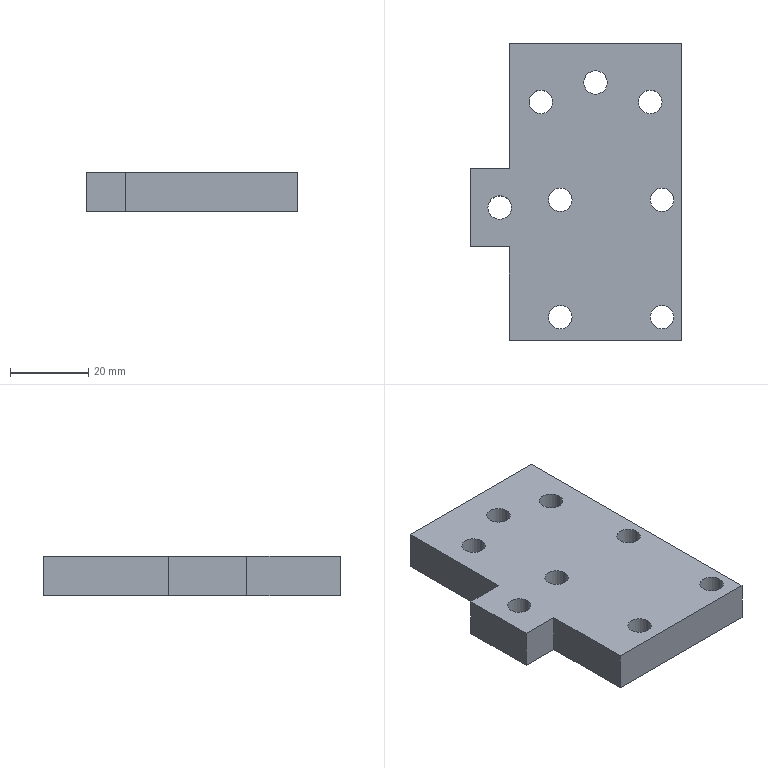Component | SolidWorks | SupportPlate-1 | 1 solid | 26 faces | box 54 x 76 x 10 mm | volume 33178 mm3 | cylinder 16 | plane 10 | commonest cylinder face diameters 6 x16
build123d program:
from build123d import *

# Parameters (mm, degrees)
SKETCH1_R           = 3
BOSS_EXTRUDE1_DEPTH = 10


with BuildPart() as part:
    # Sketch1 → Boss-Extrude1 (new body)
    with BuildSketch(Plane(origin=(0, 0, -5), x_dir=(-1, 0, 0), z_dir=(0, 0, -1))):
        Polygon((22, -9), (32, -9), (32, 11), (22, 11), (22, 43), (-22, 43), (-22, -33), (22, -33), align=None)
        with Locations(Location((0, 33, 0), (0, 0, 180))):
            Circle(SKETCH1_R, mode=Mode.SUBTRACT)
        with Locations(Location((14, 28, 0), (0, 0, 180))):
            Circle(SKETCH1_R, mode=Mode.SUBTRACT)
        with Locations(Location((9, -27, 0), (0, 0, 180))):
            Circle(SKETCH1_R, mode=Mode.SUBTRACT)
        with Locations(Location((9, 3, 0), (0, 0, 180))):
            Circle(SKETCH1_R, mode=Mode.SUBTRACT)
        with Locations(Location((-17, 3, 0), (0, 0, 180))):
            Circle(SKETCH1_R, mode=Mode.SUBTRACT)
        with Locations(Location((-17, -27, 0), (0, 0, 180))):
            Circle(SKETCH1_R, mode=Mode.SUBTRACT)
        with Locations(Location((-14, 28, 0), (0, 0, 180))):
            Circle(SKETCH1_R, mode=Mode.SUBTRACT)
        with Locations(Location((24.5, 1, 0), (0, 0, 180))):
            Circle(SKETCH1_R, mode=Mode.SUBTRACT)
    extrude(amount=-BOSS_EXTRUDE1_DEPTH)


solid = part.part

# Placed as in the assembly
solid = solid.moved(Location((196.793, 568, -207.5), (0, 0, 0)))
STEP:
#1=COLOUR_RGB('',0.7922,0.8196,0.9333);
#2=FILL_AREA_STYLE_COLOUR('',#1);
#3=FILL_AREA_STYLE('',(#2));
#4=SURFACE_STYLE_FILL_AREA(#3);
#5=SURFACE_SIDE_STYLE('',(#4));
#6=SURFACE_STYLE_USAGE(.BOTH.,#5);
#7=PRESENTATION_STYLE_ASSIGNMENT((#6));
#8=CARTESIAN_POINT('',(6.901,22.402,-7.972));
#9=VERTEX_POINT('',#8);
#10=CARTESIAN_POINT('',(6.665,22.402,-7.972));
#11=VERTEX_POINT('',#10);
#12=CARTESIAN_POINT('',(6.783,22.402,-7.972));
#13=DIRECTION('',(0.,0.,-1.));
#14=DIRECTION('',(1.,0.,0.));
#15=AXIS2_PLACEMENT_3D('',#12,#13,#14);
#16=CIRCLE('',#15,0.1181);
#17=EDGE_CURVE('',#9,#11,#16,.T.);
#18=ORIENTED_EDGE('',*,*,#17,.F.);
#19=CARTESIAN_POINT('',(6.901,22.402,-8.366));
#20=VERTEX_POINT('',#19);
#21=CARTESIAN_POINT('',(6.901,22.402,-7.972));
#22=DIRECTION('',(0.,0.,-1.));
#23=VECTOR('',#22,39.37);
#24=LINE('',#21,#23);
#25=EDGE_CURVE('',#9,#20,#24,.T.);
#26=ORIENTED_EDGE('',*,*,#25,.T.);
#27=CARTESIAN_POINT('',(6.665,22.402,-8.366));
#28=VERTEX_POINT('',#27);
#29=CARTESIAN_POINT('',(6.783,22.402,-8.366));
#30=DIRECTION('',(0.,0.,-1.));
#31=DIRECTION('',(1.,0.,0.));
#32=AXIS2_PLACEMENT_3D('',#29,#30,#31);
#33=CIRCLE('',#32,0.1181);
#34=EDGE_CURVE('',#20,#28,#33,.T.);
#35=ORIENTED_EDGE('',*,*,#34,.T.);
#36=CARTESIAN_POINT('',(6.665,22.402,-7.972));
#37=DIRECTION('',(0.,0.,-1.));
#38=VECTOR('',#37,39.37);
#39=LINE('',#36,#38);
#40=EDGE_CURVE('',#11,#28,#39,.T.);
#41=ORIENTED_EDGE('',*,*,#40,.F.);
#42=EDGE_LOOP('',(#18,#26,#35,#41));
#43=FACE_OUTER_BOUND('',#42,.T.);
#44=CARTESIAN_POINT('',(6.783,22.402,-7.972));
#45=DIRECTION('',(0.,0.,-1.));
#46=DIRECTION('',(-1.,0.,0.));
#47=AXIS2_PLACEMENT_3D('',#44,#45,#46);
#48=CYLINDRICAL_SURFACE('',#47,0.1181);
#49=ADVANCED_FACE('',(#43),#48,.F.);
#50=CARTESIAN_POINT('',(8.417,23.465,-7.972));
#51=VERTEX_POINT('',#50);
#52=CARTESIAN_POINT('',(8.181,23.465,-7.972));
#53=VERTEX_POINT('',#52);
#54=CARTESIAN_POINT('',(8.299,23.465,-7.972));
#55=DIRECTION('',(0.,0.,-1.));
#56=DIRECTION('',(1.,0.,0.));
#57=AXIS2_PLACEMENT_3D('',#54,#55,#56);
#58=CIRCLE('',#57,0.1181);
#59=EDGE_CURVE('',#51,#53,#58,.T.);
#60=ORIENTED_EDGE('',*,*,#59,.F.);
#61=CARTESIAN_POINT('',(8.417,23.465,-8.366));
#62=VERTEX_POINT('',#61);
#63=CARTESIAN_POINT('',(8.417,23.465,-7.972));
#64=DIRECTION('',(0.,0.,-1.));
#65=VECTOR('',#64,39.37);
#66=LINE('',#63,#65);
#67=EDGE_CURVE('',#51,#62,#66,.T.);
#68=ORIENTED_EDGE('',*,*,#67,.T.);
#69=CARTESIAN_POINT('',(8.181,23.465,-8.366));
#70=VERTEX_POINT('',#69);
#71=CARTESIAN_POINT('',(8.299,23.465,-8.366));
#72=DIRECTION('',(0.,0.,-1.));
#73=DIRECTION('',(1.,0.,0.));
#74=AXIS2_PLACEMENT_3D('',#71,#72,#73);
#75=CIRCLE('',#74,0.1181);
#76=EDGE_CURVE('',#62,#70,#75,.T.);
#77=ORIENTED_EDGE('',*,*,#76,.T.);
#78=CARTESIAN_POINT('',(8.181,23.465,-7.972));
#79=DIRECTION('',(0.,0.,-1.));
#80=VECTOR('',#79,39.37);
#81=LINE('',#78,#80);
#82=EDGE_CURVE('',#53,#70,#81,.T.);
#83=ORIENTED_EDGE('',*,*,#82,.F.);
#84=EDGE_LOOP('',(#60,#68,#77,#83));
#85=FACE_OUTER_BOUND('',#84,.T.);
#86=CARTESIAN_POINT('',(8.299,23.465,-7.972));
#87=DIRECTION('',(0.,0.,-1.));
#88=DIRECTION('',(-1.,0.,0.));
#89=AXIS2_PLACEMENT_3D('',#86,#87,#88);
#90=CYLINDRICAL_SURFACE('',#89,0.1181);
#91=ADVANCED_FACE('',(#85),#90,.F.);
#92=CARTESIAN_POINT('',(8.535,21.299,-7.972));
#93=VERTEX_POINT('',#92);
#94=CARTESIAN_POINT('',(8.299,21.299,-7.972));
#95=VERTEX_POINT('',#94);
#96=CARTESIAN_POINT('',(8.417,21.299,-7.972));
#97=DIRECTION('',(0.,0.,-1.));
#98=DIRECTION('',(1.,0.,0.));
#99=AXIS2_PLACEMENT_3D('',#96,#97,#98);
#100=CIRCLE('',#99,0.1181);
#101=EDGE_CURVE('',#93,#95,#100,.T.);
#102=ORIENTED_EDGE('',*,*,#101,.F.);
#103=CARTESIAN_POINT('',(8.535,21.299,-8.366));
#104=VERTEX_POINT('',#103);
#105=CARTESIAN_POINT('',(8.535,21.299,-7.972));
#106=DIRECTION('',(0.,0.,-1.));
#107=VECTOR('',#106,39.37);
#108=LINE('',#105,#107);
#109=EDGE_CURVE('',#93,#104,#108,.T.);
#110=ORIENTED_EDGE('',*,*,#109,.T.);
#111=CARTESIAN_POINT('',(8.299,21.299,-8.366));
#112=VERTEX_POINT('',#111);
#113=CARTESIAN_POINT('',(8.417,21.299,-8.366));
#114=DIRECTION('',(0.,0.,-1.));
#115=DIRECTION('',(1.,0.,0.));
#116=AXIS2_PLACEMENT_3D('',#113,#114,#115);
#117=CIRCLE('',#116,0.1181);
#118=EDGE_CURVE('',#104,#112,#117,.T.);
#119=ORIENTED_EDGE('',*,*,#118,.T.);
#120=CARTESIAN_POINT('',(8.299,21.299,-7.972));
#121=DIRECTION('',(0.,0.,-1.));
#122=VECTOR('',#121,39.37);
#123=LINE('',#120,#122);
#124=EDGE_CURVE('',#95,#112,#123,.T.);
#125=ORIENTED_EDGE('',*,*,#124,.F.);
#126=EDGE_LOOP('',(#102,#110,#119,#125));
#127=FACE_OUTER_BOUND('',#126,.T.);
#128=CARTESIAN_POINT('',(8.417,21.299,-7.972));
#129=DIRECTION('',(0.,0.,-1.));
#130=DIRECTION('',(-1.,0.,0.));
#131=AXIS2_PLACEMENT_3D('',#128,#129,#130);
#132=CYLINDRICAL_SURFACE('',#131,0.1181);
#133=ADVANCED_FACE('',(#127),#132,.F.);
#134=CARTESIAN_POINT('',(8.535,22.48,-7.972));
#135=VERTEX_POINT('',#134);
#136=CARTESIAN_POINT('',(8.299,22.48,-7.972));
#137=VERTEX_POINT('',#136);
#138=CARTESIAN_POINT('',(8.417,22.48,-7.972));
#139=DIRECTION('',(0.,0.,-1.));
#140=DIRECTION('',(1.,0.,0.));
#141=AXIS2_PLACEMENT_3D('',#138,#139,#140);
#142=CIRCLE('',#141,0.1181);
#143=EDGE_CURVE('',#135,#137,#142,.T.);
#144=ORIENTED_EDGE('',*,*,#143,.F.);
#145=CARTESIAN_POINT('',(8.535,22.48,-8.366));
#146=VERTEX_POINT('',#145);
#147=CARTESIAN_POINT('',(8.535,22.48,-7.972));
#148=DIRECTION('',(0.,0.,-1.));
#149=VECTOR('',#148,39.37);
#150=LINE('',#147,#149);
#151=EDGE_CURVE('',#135,#146,#150,.T.);
#152=ORIENTED_EDGE('',*,*,#151,.T.);
#153=CARTESIAN_POINT('',(8.299,22.48,-8.366));
#154=VERTEX_POINT('',#153);
#155=CARTESIAN_POINT('',(8.417,22.48,-8.366));
#156=DIRECTION('',(0.,0.,-1.));
#157=DIRECTION('',(1.,0.,0.));
#158=AXIS2_PLACEMENT_3D('',#155,#156,#157);
#159=CIRCLE('',#158,0.1181);
#160=EDGE_CURVE('',#146,#154,#159,.T.);
#161=ORIENTED_EDGE('',*,*,#160,.T.);
#162=CARTESIAN_POINT('',(8.299,22.48,-7.972));
#163=DIRECTION('',(0.,0.,-1.));
#164=VECTOR('',#163,39.37);
#165=LINE('',#162,#164);
#166=EDGE_CURVE('',#137,#154,#165,.T.);
#167=ORIENTED_EDGE('',*,*,#166,.F.);
#168=EDGE_LOOP('',(#144,#152,#161,#167));
#169=FACE_OUTER_BOUND('',#168,.T.);
#170=CARTESIAN_POINT('',(8.417,22.48,-7.972));
#171=DIRECTION('',(0.,0.,-1.));
#172=DIRECTION('',(-1.,0.,0.));
#173=AXIS2_PLACEMENT_3D('',#170,#171,#172);
#174=CYLINDRICAL_SURFACE('',#173,0.1181);
#175=ADVANCED_FACE('',(#169),#174,.F.);
#176=CARTESIAN_POINT('',(7.512,22.48,-7.972));
#177=VERTEX_POINT('',#176);
#178=CARTESIAN_POINT('',(7.275,22.48,-7.972));
#179=VERTEX_POINT('',#178);
#180=CARTESIAN_POINT('',(7.393,22.48,-7.972));
#181=DIRECTION('',(0.,0.,-1.));
#182=DIRECTION('',(1.,0.,0.));
#183=AXIS2_PLACEMENT_3D('',#180,#181,#182);
#184=CIRCLE('',#183,0.1181);
#185=EDGE_CURVE('',#177,#179,#184,.T.);
#186=ORIENTED_EDGE('',*,*,#185,.F.);
#187=CARTESIAN_POINT('',(7.512,22.48,-8.366));
#188=VERTEX_POINT('',#187);
#189=CARTESIAN_POINT('',(7.512,22.48,-7.972));
#190=DIRECTION('',(0.,0.,-1.));
#191=VECTOR('',#190,39.37);
#192=LINE('',#189,#191);
#193=EDGE_CURVE('',#177,#188,#192,.T.);
#194=ORIENTED_EDGE('',*,*,#193,.T.);
#195=CARTESIAN_POINT('',(7.275,22.48,-8.366));
#196=VERTEX_POINT('',#195);
#197=CARTESIAN_POINT('',(7.393,22.48,-8.366));
#198=DIRECTION('',(0.,0.,-1.));
#199=DIRECTION('',(1.,0.,0.));
#200=AXIS2_PLACEMENT_3D('',#197,#198,#199);
#201=CIRCLE('',#200,0.1181);
#202=EDGE_CURVE('',#188,#196,#201,.T.);
#203=ORIENTED_EDGE('',*,*,#202,.T.);
#204=CARTESIAN_POINT('',(7.275,22.48,-7.972));
#205=DIRECTION('',(0.,0.,-1.));
#206=VECTOR('',#205,39.37);
#207=LINE('',#204,#206);
#208=EDGE_CURVE('',#179,#196,#207,.T.);
#209=ORIENTED_EDGE('',*,*,#208,.F.);
#210=EDGE_LOOP('',(#186,#194,#203,#209));
#211=FACE_OUTER_BOUND('',#210,.T.);
#212=CARTESIAN_POINT('',(7.393,22.48,-7.972));
#213=DIRECTION('',(0.,0.,-1.));
#214=DIRECTION('',(-1.,0.,0.));
#215=AXIS2_PLACEMENT_3D('',#212,#213,#214);
#216=CYLINDRICAL_SURFACE('',#215,0.1181);
#217=ADVANCED_FACE('',(#211),#216,.F.);
#218=CARTESIAN_POINT('',(7.512,21.299,-7.972));
#219=VERTEX_POINT('',#218);
#220=CARTESIAN_POINT('',(7.275,21.299,-7.972));
#221=VERTEX_POINT('',#220);
#222=CARTESIAN_POINT('',(7.393,21.299,-7.972));
#223=DIRECTION('',(0.,0.,-1.));
#224=DIRECTION('',(1.,0.,0.));
#225=AXIS2_PLACEMENT_3D('',#222,#223,#224);
#226=CIRCLE('',#225,0.1181);
#227=EDGE_CURVE('',#219,#221,#226,.T.);
#228=ORIENTED_EDGE('',*,*,#227,.F.);
#229=CARTESIAN_POINT('',(7.512,21.299,-8.366));
#230=VERTEX_POINT('',#229);
#231=CARTESIAN_POINT('',(7.512,21.299,-7.972));
#232=DIRECTION('',(0.,0.,-1.));
#233=VECTOR('',#232,39.37);
#234=LINE('',#231,#233);
#235=EDGE_CURVE('',#219,#230,#234,.T.);
#236=ORIENTED_EDGE('',*,*,#235,.T.);
#237=CARTESIAN_POINT('',(7.275,21.299,-8.366));
#238=VERTEX_POINT('',#237);
#239=CARTESIAN_POINT('',(7.393,21.299,-8.366));
#240=DIRECTION('',(0.,0.,-1.));
#241=DIRECTION('',(1.,0.,0.));
#242=AXIS2_PLACEMENT_3D('',#239,#240,#241);
#243=CIRCLE('',#242,0.1181);
#244=EDGE_CURVE('',#230,#238,#243,.T.);
#245=ORIENTED_EDGE('',*,*,#244,.T.);
#246=CARTESIAN_POINT('',(7.275,21.299,-7.972));
#247=DIRECTION('',(0.,0.,-1.));
#248=VECTOR('',#247,39.37);
#249=LINE('',#246,#248);
#250=EDGE_CURVE('',#221,#238,#249,.T.);
#251=ORIENTED_EDGE('',*,*,#250,.F.);
#252=EDGE_LOOP('',(#228,#236,#245,#251));
#253=FACE_OUTER_BOUND('',#252,.T.);
#254=CARTESIAN_POINT('',(7.393,21.299,-7.972));
#255=DIRECTION('',(0.,0.,-1.));
#256=DIRECTION('',(-1.,0.,0.));
#257=AXIS2_PLACEMENT_3D('',#254,#255,#256);
#258=CYLINDRICAL_SURFACE('',#257,0.1181);
#259=ADVANCED_FACE('',(#253),#258,.F.);
#260=CARTESIAN_POINT('',(7.315,23.465,-7.972));
#261=VERTEX_POINT('',#260);
#262=CARTESIAN_POINT('',(7.078,23.465,-7.972));
#263=VERTEX_POINT('',#262);
#264=CARTESIAN_POINT('',(7.197,23.465,-7.972));
#265=DIRECTION('',(0.,0.,-1.));
#266=DIRECTION('',(1.,0.,0.));
#267=AXIS2_PLACEMENT_3D('',#264,#265,#266);
#268=CIRCLE('',#267,0.1181);
#269=EDGE_CURVE('',#261,#263,#268,.T.);
#270=ORIENTED_EDGE('',*,*,#269,.F.);
#271=CARTESIAN_POINT('',(7.315,23.465,-8.366));
#272=VERTEX_POINT('',#271);
#273=CARTESIAN_POINT('',(7.315,23.465,-7.972));
#274=DIRECTION('',(0.,0.,-1.));
#275=VECTOR('',#274,39.37);
#276=LINE('',#273,#275);
#277=EDGE_CURVE('',#261,#272,#276,.T.);
#278=ORIENTED_EDGE('',*,*,#277,.T.);
#279=CARTESIAN_POINT('',(7.078,23.465,-8.366));
#280=VERTEX_POINT('',#279);
#281=CARTESIAN_POINT('',(7.197,23.465,-8.366));
#282=DIRECTION('',(0.,0.,-1.));
#283=DIRECTION('',(1.,0.,0.));
#284=AXIS2_PLACEMENT_3D('',#281,#282,#283);
#285=CIRCLE('',#284,0.1181);
#286=EDGE_CURVE('',#272,#280,#285,.T.);
#287=ORIENTED_EDGE('',*,*,#286,.T.);
#288=CARTESIAN_POINT('',(7.078,23.465,-7.972));
#289=DIRECTION('',(0.,0.,-1.));
#290=VECTOR('',#289,39.37);
#291=LINE('',#288,#290);
#292=EDGE_CURVE('',#263,#280,#291,.T.);
#293=ORIENTED_EDGE('',*,*,#292,.F.);
#294=EDGE_LOOP('',(#270,#278,#287,#293));
#295=FACE_OUTER_BOUND('',#294,.T.);
#296=CARTESIAN_POINT('',(7.197,23.465,-7.972));
#297=DIRECTION('',(0.,0.,-1.));
#298=DIRECTION('',(-1.,0.,0.));
#299=AXIS2_PLACEMENT_3D('',#296,#297,#298);
#300=CYLINDRICAL_SURFACE('',#299,0.1181);
#301=ADVANCED_FACE('',(#295),#300,.F.);
#302=CARTESIAN_POINT('',(7.866,23.661,-7.972));
#303=VERTEX_POINT('',#302);
#304=CARTESIAN_POINT('',(7.63,23.661,-7.972));
#305=VERTEX_POINT('',#304);
#306=CARTESIAN_POINT('',(7.748,23.661,-7.972));
#307=DIRECTION('',(0.,0.,-1.));
#308=DIRECTION('',(1.,0.,0.));
#309=AXIS2_PLACEMENT_3D('',#306,#307,#308);
#310=CIRCLE('',#309,0.1181);
#311=EDGE_CURVE('',#303,#305,#310,.T.);
#312=ORIENTED_EDGE('',*,*,#311,.F.);
#313=CARTESIAN_POINT('',(7.866,23.661,-8.366));
#314=VERTEX_POINT('',#313);
#315=CARTESIAN_POINT('',(7.866,23.661,-7.972));
#316=DIRECTION('',(0.,0.,-1.));
#317=VECTOR('',#316,39.37);
#318=LINE('',#315,#317);
#319=EDGE_CURVE('',#303,#314,#318,.T.);
#320=ORIENTED_EDGE('',*,*,#319,.T.);
#321=CARTESIAN_POINT('',(7.63,23.661,-8.366));
#322=VERTEX_POINT('',#321);
#323=CARTESIAN_POINT('',(7.748,23.661,-8.366));
#324=DIRECTION('',(0.,0.,-1.));
#325=DIRECTION('',(1.,0.,0.));
#326=AXIS2_PLACEMENT_3D('',#323,#324,#325);
#327=CIRCLE('',#326,0.1181);
#328=EDGE_CURVE('',#314,#322,#327,.T.);
#329=ORIENTED_EDGE('',*,*,#328,.T.);
#330=CARTESIAN_POINT('',(7.63,23.661,-7.972));
#331=DIRECTION('',(0.,0.,-1.));
#332=VECTOR('',#331,39.37);
#333=LINE('',#330,#332);
#334=EDGE_CURVE('',#305,#322,#333,.T.);
#335=ORIENTED_EDGE('',*,*,#334,.F.);
#336=EDGE_LOOP('',(#312,#320,#329,#335));
#337=FACE_OUTER_BOUND('',#336,.T.);
#338=CARTESIAN_POINT('',(7.748,23.661,-7.972));
#339=DIRECTION('',(0.,0.,-1.));
#340=DIRECTION('',(-1.,0.,0.));
#341=AXIS2_PLACEMENT_3D('',#338,#339,#340);
#342=CYLINDRICAL_SURFACE('',#341,0.1181);
#343=ADVANCED_FACE('',(#337),#342,.F.);
#344=CARTESIAN_POINT('',(6.882,21.063,-8.366));
#345=VERTEX_POINT('',#344);
#346=CARTESIAN_POINT('',(6.882,22.008,-8.366));
#347=VERTEX_POINT('',#346);
#348=CARTESIAN_POINT('',(6.882,21.063,-8.366));
#349=DIRECTION('',(0.,1.,0.));
#350=VECTOR('',#349,39.37);
#351=LINE('',#348,#350);
#352=EDGE_CURVE('',#345,#347,#351,.T.);
#353=ORIENTED_EDGE('',*,*,#352,.F.);
#354=CARTESIAN_POINT('',(6.882,21.063,-7.972));
#355=VERTEX_POINT('',#354);
#356=CARTESIAN_POINT('',(6.882,21.063,-7.972));
#357=DIRECTION('',(0.,0.,-1.));
#358=VECTOR('',#357,39.37);
#359=LINE('',#356,#358);
#360=EDGE_CURVE('',#355,#345,#359,.T.);
#361=ORIENTED_EDGE('',*,*,#360,.F.);
#362=CARTESIAN_POINT('',(6.882,22.008,-7.972));
#363=VERTEX_POINT('',#362);
#364=CARTESIAN_POINT('',(6.882,21.063,-7.972));
#365=DIRECTION('',(0.,1.,0.));
#366=VECTOR('',#365,39.37);
#367=LINE('',#364,#366);
#368=EDGE_CURVE('',#355,#363,#367,.T.);
#369=ORIENTED_EDGE('',*,*,#368,.T.);
#370=CARTESIAN_POINT('',(6.882,22.008,-7.972));
#371=DIRECTION('',(0.,0.,-1.));
#372=VECTOR('',#371,39.37);
#373=LINE('',#370,#372);
#374=EDGE_CURVE('',#363,#347,#373,.T.);
#375=ORIENTED_EDGE('',*,*,#374,.T.);
#376=EDGE_LOOP('',(#353,#361,#369,#375));
#377=FACE_OUTER_BOUND('',#376,.T.);
#378=CARTESIAN_POINT('',(6.882,21.063,-7.972));
#379=DIRECTION('',(-1.,0.,0.));
#380=DIRECTION('',(0.,0.,1.));
#381=AXIS2_PLACEMENT_3D('',#378,#379,#380);
#382=PLANE('',#381);
#383=ADVANCED_FACE('',(#377),#382,.T.);
#384=CARTESIAN_POINT('',(8.614,21.063,-8.366));
#385=VERTEX_POINT('',#384);
#386=CARTESIAN_POINT('',(8.614,21.063,-8.366));
#387=DIRECTION('',(-1.,0.,0.));
#388=VECTOR('',#387,39.37);
#389=LINE('',#386,#388);
#390=EDGE_CURVE('',#385,#345,#389,.T.);
#391=ORIENTED_EDGE('',*,*,#390,.F.);
#392=CARTESIAN_POINT('',(8.614,21.063,-7.972));
#393=VERTEX_POINT('',#392);
#394=CARTESIAN_POINT('',(8.614,21.063,-7.972));
#395=DIRECTION('',(0.,0.,-1.));
#396=VECTOR('',#395,39.37);
#397=LINE('',#394,#396);
#398=EDGE_CURVE('',#393,#385,#397,.T.);
#399=ORIENTED_EDGE('',*,*,#398,.F.);
#400=CARTESIAN_POINT('',(8.614,21.063,-7.972));
#401=DIRECTION('',(-1.,0.,0.));
#402=VECTOR('',#401,39.37);
#403=LINE('',#400,#402);
#404=EDGE_CURVE('',#393,#355,#403,.T.);
#405=ORIENTED_EDGE('',*,*,#404,.T.);
#406=ORIENTED_EDGE('',*,*,#360,.T.);
#407=EDGE_LOOP('',(#391,#399,#405,#406));
#408=FACE_OUTER_BOUND('',#407,.T.);
#409=CARTESIAN_POINT('',(8.614,21.063,-7.972));
#410=DIRECTION('',(0.,-1.,0.));
#411=DIRECTION('',(0.,0.,-1.));
#412=AXIS2_PLACEMENT_3D('',#409,#410,#411);
#413=PLANE('',#412);
#414=ADVANCED_FACE('',(#408),#413,.T.);
#415=CARTESIAN_POINT('',(8.614,24.055,-8.366));
#416=VERTEX_POINT('',#415);
#417=CARTESIAN_POINT('',(8.614,24.055,-8.366));
#418=DIRECTION('',(0.,-1.,0.));
#419=VECTOR('',#418,39.37);
#420=LINE('',#417,#419);
#421=EDGE_CURVE('',#416,#385,#420,.T.);
#422=ORIENTED_EDGE('',*,*,#421,.F.);
#423=CARTESIAN_POINT('',(8.614,24.055,-7.972));
#424=VERTEX_POINT('',#423);
#425=CARTESIAN_POINT('',(8.614,24.055,-7.972));
#426=DIRECTION('',(0.,0.,-1.));
#427=VECTOR('',#426,39.37);
#428=LINE('',#425,#427);
#429=EDGE_CURVE('',#424,#416,#428,.T.);
#430=ORIENTED_EDGE('',*,*,#429,.F.);
#431=CARTESIAN_POINT('',(8.614,24.055,-7.972));
#432=DIRECTION('',(0.,-1.,0.));
#433=VECTOR('',#432,39.37);
#434=LINE('',#431,#433);
#435=EDGE_CURVE('',#424,#393,#434,.T.);
#436=ORIENTED_EDGE('',*,*,#435,.T.);
#437=ORIENTED_EDGE('',*,*,#398,.T.);
#438=EDGE_LOOP('',(#422,#430,#436,#437));
#439=FACE_OUTER_BOUND('',#438,.T.);
#440=CARTESIAN_POINT('',(8.614,24.055,-7.972));
#441=DIRECTION('',(1.,0.,0.));
#442=DIRECTION('',(0.,0.,-1.));
#443=AXIS2_PLACEMENT_3D('',#440,#441,#442);
#444=PLANE('',#443);
#445=ADVANCED_FACE('',(#439),#444,.T.);
#446=CARTESIAN_POINT('',(6.882,24.055,-8.366));
#447=VERTEX_POINT('',#446);
#448=CARTESIAN_POINT('',(6.882,24.055,-8.366));
#449=DIRECTION('',(1.,0.,0.));
#450=VECTOR('',#449,39.37);
#451=LINE('',#448,#450);
#452=EDGE_CURVE('',#447,#416,#451,.T.);
#453=ORIENTED_EDGE('',*,*,#452,.F.);
#454=CARTESIAN_POINT('',(6.882,24.055,-7.972));
#455=VERTEX_POINT('',#454);
#456=CARTESIAN_POINT('',(6.882,24.055,-7.972));
#457=DIRECTION('',(0.,0.,-1.));
#458=VECTOR('',#457,39.37);
#459=LINE('',#456,#458);
#460=EDGE_CURVE('',#455,#447,#459,.T.);
#461=ORIENTED_EDGE('',*,*,#460,.F.);
#462=CARTESIAN_POINT('',(6.882,24.055,-7.972));
#463=DIRECTION('',(1.,0.,0.));
#464=VECTOR('',#463,39.37);
#465=LINE('',#462,#464);
#466=EDGE_CURVE('',#455,#424,#465,.T.);
#467=ORIENTED_EDGE('',*,*,#466,.T.);
#468=ORIENTED_EDGE('',*,*,#429,.T.);
#469=EDGE_LOOP('',(#453,#461,#467,#468));
#470=FACE_OUTER_BOUND('',#469,.T.);
#471=CARTESIAN_POINT('',(6.882,24.055,-7.972));
#472=DIRECTION('',(-0.,1.,0.));
#473=DIRECTION('',(-1.,-0.,0.));
#474=AXIS2_PLACEMENT_3D('',#471,#472,#473);
#475=PLANE('',#474);
#476=ADVANCED_FACE('',(#470),#475,.T.);
#477=CARTESIAN_POINT('',(6.882,22.795,-8.366));
#478=VERTEX_POINT('',#477);
#479=CARTESIAN_POINT('',(6.882,22.795,-8.366));
#480=DIRECTION('',(0.,1.,0.));
#481=VECTOR('',#480,39.37);
#482=LINE('',#479,#481);
#483=EDGE_CURVE('',#478,#447,#482,.T.);
#484=ORIENTED_EDGE('',*,*,#483,.F.);
#485=CARTESIAN_POINT('',(6.882,22.795,-7.972));
#486=VERTEX_POINT('',#485);
#487=CARTESIAN_POINT('',(6.882,22.795,-7.972));
#488=DIRECTION('',(0.,0.,-1.));
#489=VECTOR('',#488,39.37);
#490=LINE('',#487,#489);
#491=EDGE_CURVE('',#486,#478,#490,.T.);
#492=ORIENTED_EDGE('',*,*,#491,.F.);
#493=CARTESIAN_POINT('',(6.882,22.795,-7.972));
#494=DIRECTION('',(0.,1.,0.));
#495=VECTOR('',#494,39.37);
#496=LINE('',#493,#495);
#497=EDGE_CURVE('',#486,#455,#496,.T.);
#498=ORIENTED_EDGE('',*,*,#497,.T.);
#499=ORIENTED_EDGE('',*,*,#460,.T.);
#500=EDGE_LOOP('',(#484,#492,#498,#499));
#501=FACE_OUTER_BOUND('',#500,.T.);
#502=CARTESIAN_POINT('',(6.882,22.795,-7.972));
#503=DIRECTION('',(-1.,0.,0.));
#504=DIRECTION('',(0.,0.,1.));
#505=AXIS2_PLACEMENT_3D('',#502,#503,#504);
#506=PLANE('',#505);
#507=ADVANCED_FACE('',(#501),#506,.T.);
#508=CARTESIAN_POINT('',(6.488,22.795,-8.366));
#509=VERTEX_POINT('',#508);
#510=CARTESIAN_POINT('',(6.488,22.795,-8.366));
#511=DIRECTION('',(1.,0.,0.));
#512=VECTOR('',#511,39.37);
#513=LINE('',#510,#512);
#514=EDGE_CURVE('',#509,#478,#513,.T.);
#515=ORIENTED_EDGE('',*,*,#514,.F.);
#516=CARTESIAN_POINT('',(6.488,22.795,-7.972));
#517=VERTEX_POINT('',#516);
#518=CARTESIAN_POINT('',(6.488,22.795,-7.972));
#519=DIRECTION('',(0.,0.,-1.));
#520=VECTOR('',#519,39.37);
#521=LINE('',#518,#520);
#522=EDGE_CURVE('',#517,#509,#521,.T.);
#523=ORIENTED_EDGE('',*,*,#522,.F.);
#524=CARTESIAN_POINT('',(6.488,22.795,-7.972));
#525=DIRECTION('',(1.,0.,0.));
#526=VECTOR('',#525,39.37);
#527=LINE('',#524,#526);
#528=EDGE_CURVE('',#517,#486,#527,.T.);
#529=ORIENTED_EDGE('',*,*,#528,.T.);
#530=ORIENTED_EDGE('',*,*,#491,.T.);
#531=EDGE_LOOP('',(#515,#523,#529,#530));
#532=FACE_OUTER_BOUND('',#531,.T.);
#533=CARTESIAN_POINT('',(6.488,22.795,-7.972));
#534=DIRECTION('',(-0.,1.,0.));
#535=DIRECTION('',(-1.,-0.,0.));
#536=AXIS2_PLACEMENT_3D('',#533,#534,#535);
#537=PLANE('',#536);
#538=ADVANCED_FACE('',(#532),#537,.T.);
#539=CARTESIAN_POINT('',(6.488,22.008,-8.366));
#540=VERTEX_POINT('',#539);
#541=CARTESIAN_POINT('',(6.488,22.008,-8.366));
#542=DIRECTION('',(0.,1.,0.));
#543=VECTOR('',#542,39.37);
#544=LINE('',#541,#543);
#545=EDGE_CURVE('',#540,#509,#544,.T.);
#546=ORIENTED_EDGE('',*,*,#545,.F.);
#547=CARTESIAN_POINT('',(6.488,22.008,-7.972));
#548=VERTEX_POINT('',#547);
#549=CARTESIAN_POINT('',(6.488,22.008,-7.972));
#550=DIRECTION('',(0.,0.,-1.));
#551=VECTOR('',#550,39.37);
#552=LINE('',#549,#551);
#553=EDGE_CURVE('',#548,#540,#552,.T.);
#554=ORIENTED_EDGE('',*,*,#553,.F.);
#555=CARTESIAN_POINT('',(6.488,22.008,-7.972));
#556=DIRECTION('',(0.,1.,0.));
#557=VECTOR('',#556,39.37);
#558=LINE('',#555,#557);
#559=EDGE_CURVE('',#548,#517,#558,.T.);
#560=ORIENTED_EDGE('',*,*,#559,.T.);
#561=ORIENTED_EDGE('',*,*,#522,.T.);
#562=EDGE_LOOP('',(#546,#554,#560,#561));
#563=FACE_OUTER_BOUND('',#562,.T.);
#564=CARTESIAN_POINT('',(6.488,22.008,-7.972));
#565=DIRECTION('',(-1.,0.,0.));
#566=DIRECTION('',(0.,0.,1.));
#567=AXIS2_PLACEMENT_3D('',#564,#565,#566);
#568=PLANE('',#567);
#569=ADVANCED_FACE('',(#563),#568,.T.);
#570=CARTESIAN_POINT('',(6.882,22.008,-8.366));
#571=DIRECTION('',(-1.,0.,0.));
#572=VECTOR('',#571,39.37);
#573=LINE('',#570,#572);
#574=EDGE_CURVE('',#347,#540,#573,.T.);
#575=ORIENTED_EDGE('',*,*,#574,.F.);
#576=ORIENTED_EDGE('',*,*,#374,.F.);
#577=CARTESIAN_POINT('',(6.882,22.008,-7.972));
#578=DIRECTION('',(-1.,0.,0.));
#579=VECTOR('',#578,39.37);
#580=LINE('',#577,#579);
#581=EDGE_CURVE('',#363,#548,#580,.T.);
#582=ORIENTED_EDGE('',*,*,#581,.T.);
#583=ORIENTED_EDGE('',*,*,#553,.T.);
#584=EDGE_LOOP('',(#575,#576,#582,#583));
#585=FACE_OUTER_BOUND('',#584,.T.);
#586=CARTESIAN_POINT('',(6.882,22.008,-7.972));
#587=DIRECTION('',(0.,-1.,0.));
#588=DIRECTION('',(0.,0.,-1.));
#589=AXIS2_PLACEMENT_3D('',#586,#587,#588);
#590=PLANE('',#589);
#591=ADVANCED_FACE('',(#585),#590,.T.);
#592=CARTESIAN_POINT('',(6.783,22.402,-7.972));
#593=DIRECTION('',(0.,0.,-1.));
#594=DIRECTION('',(1.,0.,0.));
#595=AXIS2_PLACEMENT_3D('',#592,#593,#594);
#596=CIRCLE('',#595,0.1181);
#597=EDGE_CURVE('',#11,#9,#596,.T.);
#598=ORIENTED_EDGE('',*,*,#597,.T.);
#599=ORIENTED_EDGE('',*,*,#17,.T.);
#600=EDGE_LOOP('',(#598,#599));
#601=FACE_BOUND('',#600,.T.);
#602=CARTESIAN_POINT('',(8.299,23.465,-7.972));
#603=DIRECTION('',(0.,0.,-1.));
#604=DIRECTION('',(1.,0.,0.));
#605=AXIS2_PLACEMENT_3D('',#602,#603,#604);
#606=CIRCLE('',#605,0.1181);
#607=EDGE_CURVE('',#53,#51,#606,.T.);
#608=ORIENTED_EDGE('',*,*,#607,.T.);
#609=ORIENTED_EDGE('',*,*,#59,.T.);
#610=EDGE_LOOP('',(#608,#609));
#611=FACE_BOUND('',#610,.T.);
#612=CARTESIAN_POINT('',(8.417,21.299,-7.972));
#613=DIRECTION('',(0.,0.,-1.));
#614=DIRECTION('',(1.,0.,0.));
#615=AXIS2_PLACEMENT_3D('',#612,#613,#614);
#616=CIRCLE('',#615,0.1181);
#617=EDGE_CURVE('',#95,#93,#616,.T.);
#618=ORIENTED_EDGE('',*,*,#617,.T.);
#619=ORIENTED_EDGE('',*,*,#101,.T.);
#620=EDGE_LOOP('',(#618,#619));
#621=FACE_BOUND('',#620,.T.);
#622=CARTESIAN_POINT('',(8.417,22.48,-7.972));
#623=DIRECTION('',(0.,0.,-1.));
#624=DIRECTION('',(1.,0.,0.));
#625=AXIS2_PLACEMENT_3D('',#622,#623,#624);
#626=CIRCLE('',#625,0.1181);
#627=EDGE_CURVE('',#137,#135,#626,.T.);
#628=ORIENTED_EDGE('',*,*,#627,.T.);
#629=ORIENTED_EDGE('',*,*,#143,.T.);
#630=EDGE_LOOP('',(#628,#629));
#631=FACE_BOUND('',#630,.T.);
#632=CARTESIAN_POINT('',(7.393,22.48,-7.972));
#633=DIRECTION('',(0.,0.,-1.));
#634=DIRECTION('',(1.,0.,0.));
#635=AXIS2_PLACEMENT_3D('',#632,#633,#634);
#636=CIRCLE('',#635,0.1181);
#637=EDGE_CURVE('',#179,#177,#636,.T.);
#638=ORIENTED_EDGE('',*,*,#637,.T.);
#639=ORIENTED_EDGE('',*,*,#185,.T.);
#640=EDGE_LOOP('',(#638,#639));
#641=FACE_BOUND('',#640,.T.);
#642=CARTESIAN_POINT('',(7.393,21.299,-7.972));
#643=DIRECTION('',(0.,0.,-1.));
#644=DIRECTION('',(1.,0.,0.));
#645=AXIS2_PLACEMENT_3D('',#642,#643,#644);
#646=CIRCLE('',#645,0.1181);
#647=EDGE_CURVE('',#221,#219,#646,.T.);
#648=ORIENTED_EDGE('',*,*,#647,.T.);
#649=ORIENTED_EDGE('',*,*,#227,.T.);
#650=EDGE_LOOP('',(#648,#649));
#651=FACE_BOUND('',#650,.T.);
#652=CARTESIAN_POINT('',(7.197,23.465,-7.972));
#653=DIRECTION('',(0.,0.,-1.));
#654=DIRECTION('',(1.,0.,0.));
#655=AXIS2_PLACEMENT_3D('',#652,#653,#654);
#656=CIRCLE('',#655,0.1181);
#657=EDGE_CURVE('',#263,#261,#656,.T.);
#658=ORIENTED_EDGE('',*,*,#657,.T.);
#659=ORIENTED_EDGE('',*,*,#269,.T.);
#660=EDGE_LOOP('',(#658,#659));
#661=FACE_BOUND('',#660,.T.);
#662=CARTESIAN_POINT('',(7.748,23.661,-7.972));
#663=DIRECTION('',(0.,0.,-1.));
#664=DIRECTION('',(1.,0.,0.));
#665=AXIS2_PLACEMENT_3D('',#662,#663,#664);
#666=CIRCLE('',#665,0.1181);
#667=EDGE_CURVE('',#305,#303,#666,.T.);
#668=ORIENTED_EDGE('',*,*,#667,.T.);
#669=ORIENTED_EDGE('',*,*,#311,.T.);
#670=EDGE_LOOP('',(#668,#669));
#671=FACE_BOUND('',#670,.T.);
#672=ORIENTED_EDGE('',*,*,#368,.F.);
#673=ORIENTED_EDGE('',*,*,#404,.F.);
#674=ORIENTED_EDGE('',*,*,#435,.F.);
#675=ORIENTED_EDGE('',*,*,#466,.F.);
#676=ORIENTED_EDGE('',*,*,#497,.F.);
#677=ORIENTED_EDGE('',*,*,#528,.F.);
#678=ORIENTED_EDGE('',*,*,#559,.F.);
#679=ORIENTED_EDGE('',*,*,#581,.F.);
#680=EDGE_LOOP('',(#672,#673,#674,#675,#676,#677,#678,#679));
#681=FACE_OUTER_BOUND('',#680,.T.);
#682=CARTESIAN_POINT('',(7.748,22.362,-7.972));
#683=DIRECTION('',(0.,0.,1.));
#684=DIRECTION('',(1.,0.,0.));
#685=AXIS2_PLACEMENT_3D('',#682,#683,#684);
#686=PLANE('',#685);
#687=ADVANCED_FACE('',(#601,#611,#621,#631,#641,#651,#661,#671,#681),#686,.T.);
#688=CARTESIAN_POINT('',(6.783,22.402,-8.366));
#689=DIRECTION('',(0.,0.,-1.));
#690=DIRECTION('',(1.,0.,0.));
#691=AXIS2_PLACEMENT_3D('',#688,#689,#690);
#692=CIRCLE('',#691,0.1181);
#693=EDGE_CURVE('',#28,#20,#692,.T.);
#694=ORIENTED_EDGE('',*,*,#693,.F.);
#695=ORIENTED_EDGE('',*,*,#34,.F.);
#696=EDGE_LOOP('',(#694,#695));
#697=FACE_BOUND('',#696,.T.);
#698=CARTESIAN_POINT('',(8.299,23.465,-8.366));
#699=DIRECTION('',(0.,0.,-1.));
#700=DIRECTION('',(1.,0.,0.));
#701=AXIS2_PLACEMENT_3D('',#698,#699,#700);
#702=CIRCLE('',#701,0.1181);
#703=EDGE_CURVE('',#70,#62,#702,.T.);
#704=ORIENTED_EDGE('',*,*,#703,.F.);
#705=ORIENTED_EDGE('',*,*,#76,.F.);
#706=EDGE_LOOP('',(#704,#705));
#707=FACE_BOUND('',#706,.T.);
#708=CARTESIAN_POINT('',(8.417,21.299,-8.366));
#709=DIRECTION('',(0.,0.,-1.));
#710=DIRECTION('',(1.,0.,0.));
#711=AXIS2_PLACEMENT_3D('',#708,#709,#710);
#712=CIRCLE('',#711,0.1181);
#713=EDGE_CURVE('',#112,#104,#712,.T.);
#714=ORIENTED_EDGE('',*,*,#713,.F.);
#715=ORIENTED_EDGE('',*,*,#118,.F.);
#716=EDGE_LOOP('',(#714,#715));
#717=FACE_BOUND('',#716,.T.);
#718=CARTESIAN_POINT('',(8.417,22.48,-8.366));
#719=DIRECTION('',(0.,0.,-1.));
#720=DIRECTION('',(1.,0.,0.));
#721=AXIS2_PLACEMENT_3D('',#718,#719,#720);
#722=CIRCLE('',#721,0.1181);
#723=EDGE_CURVE('',#154,#146,#722,.T.);
#724=ORIENTED_EDGE('',*,*,#723,.F.);
#725=ORIENTED_EDGE('',*,*,#160,.F.);
#726=EDGE_LOOP('',(#724,#725));
#727=FACE_BOUND('',#726,.T.);
#728=CARTESIAN_POINT('',(7.393,22.48,-8.366));
#729=DIRECTION('',(0.,0.,-1.));
#730=DIRECTION('',(1.,0.,0.));
#731=AXIS2_PLACEMENT_3D('',#728,#729,#730);
#732=CIRCLE('',#731,0.1181);
#733=EDGE_CURVE('',#196,#188,#732,.T.);
#734=ORIENTED_EDGE('',*,*,#733,.F.);
#735=ORIENTED_EDGE('',*,*,#202,.F.);
#736=EDGE_LOOP('',(#734,#735));
#737=FACE_BOUND('',#736,.T.);
#738=CARTESIAN_POINT('',(7.393,21.299,-8.366));
#739=DIRECTION('',(0.,0.,-1.));
#740=DIRECTION('',(1.,0.,0.));
#741=AXIS2_PLACEMENT_3D('',#738,#739,#740);
#742=CIRCLE('',#741,0.1181);
#743=EDGE_CURVE('',#238,#230,#742,.T.);
#744=ORIENTED_EDGE('',*,*,#743,.F.);
#745=ORIENTED_EDGE('',*,*,#244,.F.);
#746=EDGE_LOOP('',(#744,#745));
#747=FACE_BOUND('',#746,.T.);
#748=CARTESIAN_POINT('',(7.197,23.465,-8.366));
#749=DIRECTION('',(0.,0.,-1.));
#750=DIRECTION('',(1.,0.,0.));
#751=AXIS2_PLACEMENT_3D('',#748,#749,#750);
#752=CIRCLE('',#751,0.1181);
#753=EDGE_CURVE('',#280,#272,#752,.T.);
#754=ORIENTED_EDGE('',*,*,#753,.F.);
#755=ORIENTED_EDGE('',*,*,#286,.F.);
#756=EDGE_LOOP('',(#754,#755));
#757=FACE_BOUND('',#756,.T.);
#758=CARTESIAN_POINT('',(7.748,23.661,-8.366));
#759=DIRECTION('',(0.,0.,-1.));
#760=DIRECTION('',(1.,0.,0.));
#761=AXIS2_PLACEMENT_3D('',#758,#759,#760);
#762=CIRCLE('',#761,0.1181);
#763=EDGE_CURVE('',#322,#314,#762,.T.);
#764=ORIENTED_EDGE('',*,*,#763,.F.);
#765=ORIENTED_EDGE('',*,*,#328,.F.);
#766=EDGE_LOOP('',(#764,#765));
#767=FACE_BOUND('',#766,.T.);
#768=ORIENTED_EDGE('',*,*,#352,.T.);
#769=ORIENTED_EDGE('',*,*,#574,.T.);
#770=ORIENTED_EDGE('',*,*,#545,.T.);
#771=ORIENTED_EDGE('',*,*,#514,.T.);
#772=ORIENTED_EDGE('',*,*,#483,.T.);
#773=ORIENTED_EDGE('',*,*,#452,.T.);
#774=ORIENTED_EDGE('',*,*,#421,.T.);
#775=ORIENTED_EDGE('',*,*,#390,.T.);
#776=EDGE_LOOP('',(#768,#769,#770,#771,#772,#773,#774,#775));
#777=FACE_OUTER_BOUND('',#776,.T.);
#778=CARTESIAN_POINT('',(7.748,22.362,-8.366));
#779=DIRECTION('',(0.,0.,1.));
#780=DIRECTION('',(1.,0.,0.));
#781=AXIS2_PLACEMENT_3D('',#778,#779,#780);
#782=PLANE('',#781);
#783=ADVANCED_FACE('',(#697,#707,#717,#727,#737,#747,#757,#767,#777),#782,.F.);
#784=ORIENTED_EDGE('',*,*,#319,.F.);
#785=ORIENTED_EDGE('',*,*,#667,.F.);
#786=ORIENTED_EDGE('',*,*,#334,.T.);
#787=ORIENTED_EDGE('',*,*,#763,.T.);
#788=EDGE_LOOP('',(#784,#785,#786,#787));
#789=FACE_OUTER_BOUND('',#788,.T.);
#790=CARTESIAN_POINT('',(7.748,23.661,-7.972));
#791=DIRECTION('',(0.,0.,-1.));
#792=DIRECTION('',(-1.,0.,0.));
#793=AXIS2_PLACEMENT_3D('',#790,#791,#792);
#794=CYLINDRICAL_SURFACE('',#793,0.1181);
#795=ADVANCED_FACE('',(#789),#794,.F.);
#796=ORIENTED_EDGE('',*,*,#277,.F.);
#797=ORIENTED_EDGE('',*,*,#657,.F.);
#798=ORIENTED_EDGE('',*,*,#292,.T.);
#799=ORIENTED_EDGE('',*,*,#753,.T.);
#800=EDGE_LOOP('',(#796,#797,#798,#799));
#801=FACE_OUTER_BOUND('',#800,.T.);
#802=CARTESIAN_POINT('',(7.197,23.465,-7.972));
#803=DIRECTION('',(0.,0.,-1.));
#804=DIRECTION('',(-1.,0.,0.));
#805=AXIS2_PLACEMENT_3D('',#802,#803,#804);
#806=CYLINDRICAL_SURFACE('',#805,0.1181);
#807=ADVANCED_FACE('',(#801),#806,.F.);
#808=ORIENTED_EDGE('',*,*,#235,.F.);
#809=ORIENTED_EDGE('',*,*,#647,.F.);
#810=ORIENTED_EDGE('',*,*,#250,.T.);
#811=ORIENTED_EDGE('',*,*,#743,.T.);
#812=EDGE_LOOP('',(#808,#809,#810,#811));
#813=FACE_OUTER_BOUND('',#812,.T.);
#814=CARTESIAN_POINT('',(7.393,21.299,-7.972));
#815=DIRECTION('',(0.,0.,-1.));
#816=DIRECTION('',(-1.,0.,0.));
#817=AXIS2_PLACEMENT_3D('',#814,#815,#816);
#818=CYLINDRICAL_SURFACE('',#817,0.1181);
#819=ADVANCED_FACE('',(#813),#818,.F.);
#820=ORIENTED_EDGE('',*,*,#193,.F.);
#821=ORIENTED_EDGE('',*,*,#637,.F.);
#822=ORIENTED_EDGE('',*,*,#208,.T.);
#823=ORIENTED_EDGE('',*,*,#733,.T.);
#824=EDGE_LOOP('',(#820,#821,#822,#823));
#825=FACE_OUTER_BOUND('',#824,.T.);
#826=CARTESIAN_POINT('',(7.393,22.48,-7.972));
#827=DIRECTION('',(0.,0.,-1.));
#828=DIRECTION('',(-1.,0.,0.));
#829=AXIS2_PLACEMENT_3D('',#826,#827,#828);
#830=CYLINDRICAL_SURFACE('',#829,0.1181);
#831=ADVANCED_FACE('',(#825),#830,.F.);
#832=ORIENTED_EDGE('',*,*,#151,.F.);
#833=ORIENTED_EDGE('',*,*,#627,.F.);
#834=ORIENTED_EDGE('',*,*,#166,.T.);
#835=ORIENTED_EDGE('',*,*,#723,.T.);
#836=EDGE_LOOP('',(#832,#833,#834,#835));
#837=FACE_OUTER_BOUND('',#836,.T.);
#838=CARTESIAN_POINT('',(8.417,22.48,-7.972));
#839=DIRECTION('',(0.,0.,-1.));
#840=DIRECTION('',(-1.,0.,0.));
#841=AXIS2_PLACEMENT_3D('',#838,#839,#840);
#842=CYLINDRICAL_SURFACE('',#841,0.1181);
#843=ADVANCED_FACE('',(#837),#842,.F.);
#844=ORIENTED_EDGE('',*,*,#109,.F.);
#845=ORIENTED_EDGE('',*,*,#617,.F.);
#846=ORIENTED_EDGE('',*,*,#124,.T.);
#847=ORIENTED_EDGE('',*,*,#713,.T.);
#848=EDGE_LOOP('',(#844,#845,#846,#847));
#849=FACE_OUTER_BOUND('',#848,.T.);
#850=CARTESIAN_POINT('',(8.417,21.299,-7.972));
#851=DIRECTION('',(0.,0.,-1.));
#852=DIRECTION('',(-1.,0.,0.));
#853=AXIS2_PLACEMENT_3D('',#850,#851,#852);
#854=CYLINDRICAL_SURFACE('',#853,0.1181);
#855=ADVANCED_FACE('',(#849),#854,.F.);
#856=ORIENTED_EDGE('',*,*,#67,.F.);
#857=ORIENTED_EDGE('',*,*,#607,.F.);
#858=ORIENTED_EDGE('',*,*,#82,.T.);
#859=ORIENTED_EDGE('',*,*,#703,.T.);
#860=EDGE_LOOP('',(#856,#857,#858,#859));
#861=FACE_OUTER_BOUND('',#860,.T.);
#862=CARTESIAN_POINT('',(8.299,23.465,-7.972));
#863=DIRECTION('',(0.,0.,-1.));
#864=DIRECTION('',(-1.,0.,0.));
#865=AXIS2_PLACEMENT_3D('',#862,#863,#864);
#866=CYLINDRICAL_SURFACE('',#865,0.1181);
#867=ADVANCED_FACE('',(#861),#866,.F.);
#868=ORIENTED_EDGE('',*,*,#25,.F.);
#869=ORIENTED_EDGE('',*,*,#597,.F.);
#870=ORIENTED_EDGE('',*,*,#40,.T.);
#871=ORIENTED_EDGE('',*,*,#693,.T.);
#872=EDGE_LOOP('',(#868,#869,#870,#871));
#873=FACE_OUTER_BOUND('',#872,.T.);
#874=CARTESIAN_POINT('',(6.783,22.402,-7.972));
#875=DIRECTION('',(0.,0.,-1.));
#876=DIRECTION('',(-1.,0.,0.));
#877=AXIS2_PLACEMENT_3D('',#874,#875,#876);
#878=CYLINDRICAL_SURFACE('',#877,0.1181);
#879=ADVANCED_FACE('',(#873),#878,.F.);
#880=CLOSED_SHELL('',(#49,#91,#133,#175,#217,#259,#301,#343,#383,#414,#445,#476,#507,#538,#569,#591,#687,#783,#795,#807,#819,#831,#843,#855,#867,#879));
#881=MANIFOLD_SOLID_BREP('',#880);
#882=STYLED_ITEM('',(#7),#881);
#883=PRESENTATION_LAYER_ASSIGNMENT('','',(#882));
#884=CARTESIAN_POINT('',(0.,0.,0.));
#885=DIRECTION('',(0.,0.,1.));
#886=DIRECTION('',(1.,0.,0.));
#887=AXIS2_PLACEMENT_3D('',#884,#885,#886);
#888=(LENGTH_UNIT()NAMED_UNIT(*)SI_UNIT($,.METRE.));
#889=LENGTH_MEASURE_WITH_UNIT(LENGTH_MEASURE(0.0254),#888);
#890=DIMENSIONAL_EXPONENTS(1.,0.,0.,0.,0.,0.,0.);
#891=(CONVERSION_BASED_UNIT('',#889)LENGTH_UNIT()NAMED_UNIT(#890));
#892=UNCERTAINTY_MEASURE_WITH_UNIT(LENGTH_MEASURE(0.00001),#891,'','');
#893=(NAMED_UNIT(*)PLANE_ANGLE_UNIT()SI_UNIT($,.RADIAN.));
#894=(NAMED_UNIT(*)SI_UNIT($,.STERADIAN.)SOLID_ANGLE_UNIT());
#895=(GEOMETRIC_REPRESENTATION_CONTEXT(3)GLOBAL_UNCERTAINTY_ASSIGNED_CONTEXT((#892))GLOBAL_UNIT_ASSIGNED_CONTEXT((#891,#893,#894))REPRESENTATION_CONTEXT('',''));
#896=ADVANCED_BREP_SHAPE_REPRESENTATION('',(#881,#887),#895);
#897=(LENGTH_UNIT()NAMED_UNIT(*)SI_UNIT($,.METRE.));
#898=LENGTH_MEASURE_WITH_UNIT(LENGTH_MEASURE(0.0254),#897);
#899=DIMENSIONAL_EXPONENTS(1.,0.,0.,0.,0.,0.,0.);
#900=(CONVERSION_BASED_UNIT('',#898)LENGTH_UNIT()NAMED_UNIT(#899));
#901=UNCERTAINTY_MEASURE_WITH_UNIT(LENGTH_MEASURE(0.00001),#900,'','');
#902=(NAMED_UNIT(*)PLANE_ANGLE_UNIT()SI_UNIT($,.RADIAN.));
#903=(NAMED_UNIT(*)SI_UNIT($,.STERADIAN.)SOLID_ANGLE_UNIT());
#904=(GEOMETRIC_REPRESENTATION_CONTEXT(3)GLOBAL_UNCERTAINTY_ASSIGNED_CONTEXT((#901))GLOBAL_UNIT_ASSIGNED_CONTEXT((#900,#902,#903))REPRESENTATION_CONTEXT('',''));
#905=MECHANICAL_DESIGN_GEOMETRIC_PRESENTATION_REPRESENTATION('',(#882),#904);